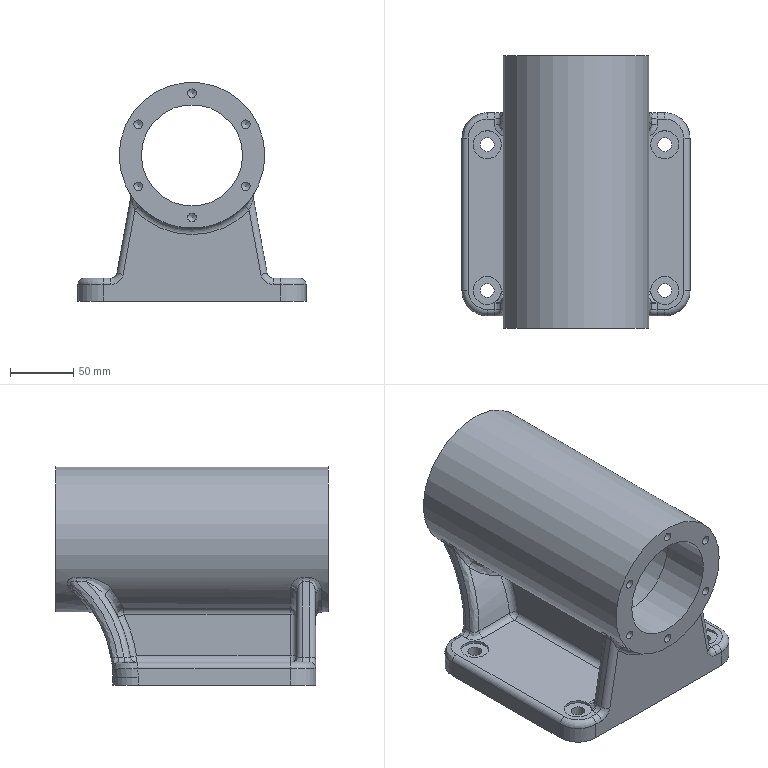Component | NX | HOUSING | 1 solid | 142 faces | volume 1681292 mm3 | cylinder 59 | spline 27 | plane 23 | torus 13 | cone 12 | sphere 8 | commonest cylinder face diameters 10 x28 6.8 x12 40 x4 11 x4 22 x4 220 x2 80 x2 115 x1